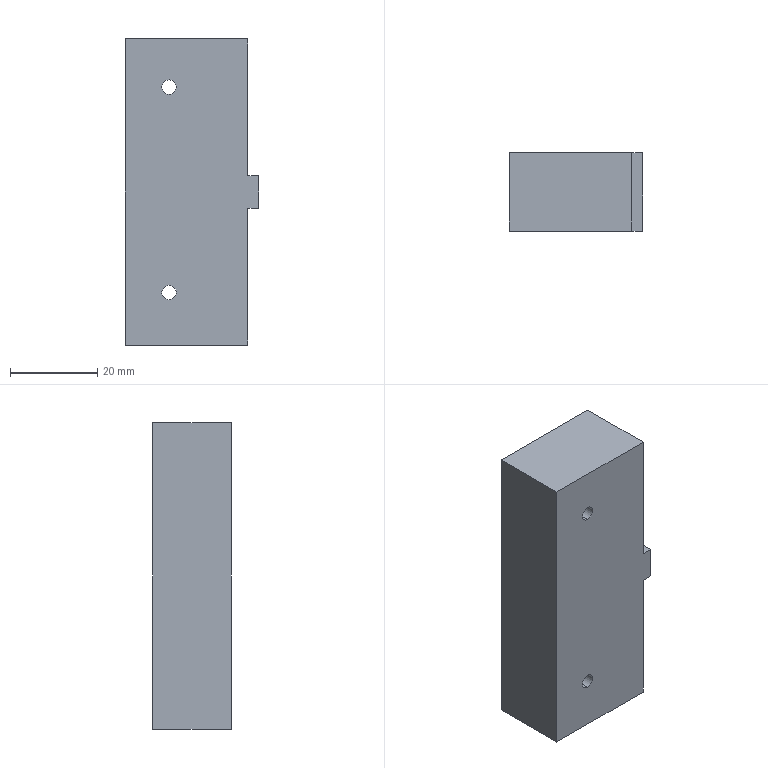Component | SolidWorks | CylinderFixingBlockS-1 | 1 solid | 22 faces | box 30.5 x 18 x 70 mm | volume 34906 mm3 | plane 10 | cylinder 8 | cone 4 | commonest cylinder face diameters 4.2 x4 3.3 x4
build123d program:
from build123d import *

# Parameters (mm, degrees)
SKETCH2_W             = 18
SKETCH2_H             = 28
BOSS_EXTRUDE1_DEPTH   = 70
M4_TAPPED_HOLE1_D     = 3.3
M5_TAPPED_HOLE1_D     = 4.2
M5_TAPPED_HOLE1_DEPTH = 14
M5_TAPPED_HOLE1_TIP   = 1.262
SKETCH8_W             = 7.4
SKETCH8_H             = 2.5
BOSS_EXTRUDE2_DEPTH   = 18


with BuildPart() as part:
    # Sketch2 → Boss-Extrude1 (new body)
    with BuildSketch(Plane.XY):
        with Locations((-28.849, -4)):
            Rectangle(SKETCH2_W, SKETCH2_H)
    extrude(amount=-BOSS_EXTRUDE1_DEPTH)

    # M4 Tapped Hole1 (through all)
    with Locations(Plane.ZY.offset(37.849)):
        with Locations((-11, 0), (-58, 0)):
            Hole(M4_TAPPED_HOLE1_D / 2)

    # M5 Tapped Hole1
    with Locations(Plane(origin=(0, -18, 0), x_dir=(-1, 0, 0), z_dir=(0, -1, 0))):
        with Locations((29.214, 58.5), (29.214, 11.5)):
            Hole(M5_TAPPED_HOLE1_D / 2, depth=M5_TAPPED_HOLE1_DEPTH)
            with Locations((0, 0, -(M5_TAPPED_HOLE1_DEPTH + M5_TAPPED_HOLE1_TIP / 2))):  # 118° drill point
                Cone(0, M5_TAPPED_HOLE1_D / 2, M5_TAPPED_HOLE1_TIP, mode=Mode.SUBTRACT)

    # Sketch8 → Boss-Extrude2 (add)
    with BuildSketch(Plane.ZY.offset(37.849)):
        with Locations((-35, -19.25)):
            Rectangle(SKETCH8_W, SKETCH8_H)
    extrude(amount=-BOSS_EXTRUDE2_DEPTH)


solid = part.part

# Placed as in the assembly
solid = solid.moved(Location((-524.996, 158.197, 306.626), (0, 0, 90)))
STEP:
#1=COLOUR_RGB('',0.7922,0.8196,0.9333);
#2=FILL_AREA_STYLE_COLOUR('',#1);
#3=FILL_AREA_STYLE('',(#2));
#4=SURFACE_STYLE_FILL_AREA(#3);
#5=SURFACE_SIDE_STYLE('',(#4));
#6=SURFACE_STYLE_USAGE(.BOTH.,#5);
#7=PRESENTATION_STYLE_ASSIGNMENT((#6));
#8=CARTESIAN_POINT('',(-20.512,5.078,9.851));
#9=VERTEX_POINT('',#8);
#10=CARTESIAN_POINT('',(-20.512,5.078,9.686));
#11=VERTEX_POINT('',#10);
#12=CARTESIAN_POINT('',(-20.512,5.078,9.769));
#13=DIRECTION('',(1.,-0.,-0.));
#14=DIRECTION('',(0.,0.,-1.));
#15=AXIS2_PLACEMENT_3D('',#12,#13,#14);
#16=CIRCLE('',#15,0.08268);
#17=EDGE_CURVE('',#9,#11,#16,.T.);
#18=ORIENTED_EDGE('',*,*,#17,.F.);
#19=CARTESIAN_POINT('',(-19.96,5.078,9.851));
#20=VERTEX_POINT('',#19);
#21=CARTESIAN_POINT('',(-19.96,5.078,9.851));
#22=DIRECTION('',(1.,-0.,-0.));
#23=VECTOR('',#22,39.37);
#24=LINE('',#21,#23);
#25=EDGE_CURVE('',#9,#20,#24,.T.);
#26=ORIENTED_EDGE('',*,*,#25,.T.);
#27=CARTESIAN_POINT('',(-19.96,5.078,9.686));
#28=VERTEX_POINT('',#27);
#29=CARTESIAN_POINT('',(-19.96,5.078,9.769));
#30=DIRECTION('',(1.,-0.,-0.));
#31=DIRECTION('',(0.,0.,-1.));
#32=AXIS2_PLACEMENT_3D('',#29,#30,#31);
#33=CIRCLE('',#32,0.08268);
#34=EDGE_CURVE('',#20,#28,#33,.T.);
#35=ORIENTED_EDGE('',*,*,#34,.T.);
#36=CARTESIAN_POINT('',(-19.96,5.078,9.686));
#37=DIRECTION('',(1.,-0.,-0.));
#38=VECTOR('',#37,39.37);
#39=LINE('',#36,#38);
#40=EDGE_CURVE('',#11,#28,#39,.T.);
#41=ORIENTED_EDGE('',*,*,#40,.F.);
#42=EDGE_LOOP('',(#18,#26,#35,#41));
#43=FACE_OUTER_BOUND('',#42,.T.);
#44=CARTESIAN_POINT('',(-19.96,5.078,9.769));
#45=DIRECTION('',(1.,-0.,-0.));
#46=DIRECTION('',(0.,0.,-1.));
#47=AXIS2_PLACEMENT_3D('',#44,#45,#46);
#48=CYLINDRICAL_SURFACE('',#47,0.08268);
#49=ADVANCED_FACE('',(#43),#48,.F.);
#50=CARTESIAN_POINT('',(-20.561,5.078,9.769));
#51=VERTEX_POINT('',#50);
#52=CARTESIAN_POINT('',(-20.512,5.078,9.686));
#53=DIRECTION('',(0.515,0.,-0.8572));
#54=VECTOR('',#53,39.37);
#55=LINE('',#52,#54);
#56=EDGE_CURVE('',#51,#11,#55,.T.);
#57=ORIENTED_EDGE('',*,*,#56,.F.);
#58=CARTESIAN_POINT('',(-20.512,5.078,9.851));
#59=DIRECTION('',(0.515,-0.,0.8572));
#60=VECTOR('',#59,39.37);
#61=LINE('',#58,#60);
#62=EDGE_CURVE('',#51,#9,#61,.T.);
#63=ORIENTED_EDGE('',*,*,#62,.T.);
#64=ORIENTED_EDGE('',*,*,#17,.T.);
#65=EDGE_LOOP('',(#57,#63,#64));
#66=FACE_OUTER_BOUND('',#65,.T.);
#67=CARTESIAN_POINT('',(-20.512,5.078,9.769));
#68=DIRECTION('',(1.,-0.,-0.));
#69=DIRECTION('',(0.,0.,-1.));
#70=AXIS2_PLACEMENT_3D('',#67,#68,#69);
#71=CONICAL_SURFACE('',#70,0.08268,1.03);
#72=ADVANCED_FACE('',(#66),#71,.F.);
#73=CARTESIAN_POINT('',(-20.512,5.078,11.702));
#74=VERTEX_POINT('',#73);
#75=CARTESIAN_POINT('',(-20.512,5.078,11.536));
#76=VERTEX_POINT('',#75);
#77=CARTESIAN_POINT('',(-20.512,5.078,11.619));
#78=DIRECTION('',(1.,-0.,-0.));
#79=DIRECTION('',(0.,0.,-1.));
#80=AXIS2_PLACEMENT_3D('',#77,#78,#79);
#81=CIRCLE('',#80,0.08268);
#82=EDGE_CURVE('',#74,#76,#81,.T.);
#83=ORIENTED_EDGE('',*,*,#82,.F.);
#84=CARTESIAN_POINT('',(-19.96,5.078,11.702));
#85=VERTEX_POINT('',#84);
#86=CARTESIAN_POINT('',(-19.96,5.078,11.702));
#87=DIRECTION('',(1.,-0.,-0.));
#88=VECTOR('',#87,39.37);
#89=LINE('',#86,#88);
#90=EDGE_CURVE('',#74,#85,#89,.T.);
#91=ORIENTED_EDGE('',*,*,#90,.T.);
#92=CARTESIAN_POINT('',(-19.96,5.078,11.536));
#93=VERTEX_POINT('',#92);
#94=CARTESIAN_POINT('',(-19.96,5.078,11.619));
#95=DIRECTION('',(1.,-0.,-0.));
#96=DIRECTION('',(0.,0.,-1.));
#97=AXIS2_PLACEMENT_3D('',#94,#95,#96);
#98=CIRCLE('',#97,0.08268);
#99=EDGE_CURVE('',#85,#93,#98,.T.);
#100=ORIENTED_EDGE('',*,*,#99,.T.);
#101=CARTESIAN_POINT('',(-19.96,5.078,11.536));
#102=DIRECTION('',(1.,-0.,-0.));
#103=VECTOR('',#102,39.37);
#104=LINE('',#101,#103);
#105=EDGE_CURVE('',#76,#93,#104,.T.);
#106=ORIENTED_EDGE('',*,*,#105,.F.);
#107=EDGE_LOOP('',(#83,#91,#100,#106));
#108=FACE_OUTER_BOUND('',#107,.T.);
#109=CARTESIAN_POINT('',(-19.96,5.078,11.619));
#110=DIRECTION('',(1.,-0.,-0.));
#111=DIRECTION('',(0.,0.,-1.));
#112=AXIS2_PLACEMENT_3D('',#109,#110,#111);
#113=CYLINDRICAL_SURFACE('',#112,0.08268);
#114=ADVANCED_FACE('',(#108),#113,.F.);
#115=CARTESIAN_POINT('',(-20.561,5.078,11.619));
#116=VERTEX_POINT('',#115);
#117=CARTESIAN_POINT('',(-20.512,5.078,11.536));
#118=DIRECTION('',(0.515,0.,-0.8572));
#119=VECTOR('',#118,39.37);
#120=LINE('',#117,#119);
#121=EDGE_CURVE('',#116,#76,#120,.T.);
#122=ORIENTED_EDGE('',*,*,#121,.F.);
#123=CARTESIAN_POINT('',(-20.512,5.078,11.702));
#124=DIRECTION('',(0.515,-0.,0.8572));
#125=VECTOR('',#124,39.37);
#126=LINE('',#123,#125);
#127=EDGE_CURVE('',#116,#74,#126,.T.);
#128=ORIENTED_EDGE('',*,*,#127,.T.);
#129=ORIENTED_EDGE('',*,*,#82,.T.);
#130=EDGE_LOOP('',(#122,#128,#129));
#131=FACE_OUTER_BOUND('',#130,.T.);
#132=CARTESIAN_POINT('',(-20.512,5.078,11.619));
#133=DIRECTION('',(1.,-0.,-0.));
#134=DIRECTION('',(0.,0.,-1.));
#135=AXIS2_PLACEMENT_3D('',#132,#133,#134);
#136=CONICAL_SURFACE('',#135,0.08268,1.03);
#137=ADVANCED_FACE('',(#131),#136,.F.);
#138=CARTESIAN_POINT('',(-20.669,5.447,11.574));
#139=VERTEX_POINT('',#138);
#140=CARTESIAN_POINT('',(-20.669,5.447,11.704));
#141=VERTEX_POINT('',#140);
#142=CARTESIAN_POINT('',(-20.669,5.447,11.639));
#143=DIRECTION('',(0.,-1.,-0.));
#144=DIRECTION('',(0.,0.,1.));
#145=AXIS2_PLACEMENT_3D('',#142,#143,#144);
#146=CIRCLE('',#145,0.06496);
#147=EDGE_CURVE('',#139,#141,#146,.T.);
#148=ORIENTED_EDGE('',*,*,#147,.F.);
#149=CARTESIAN_POINT('',(-20.669,4.738,11.574));
#150=VERTEX_POINT('',#149);
#151=CARTESIAN_POINT('',(-20.669,4.738,11.574));
#152=DIRECTION('',(0.,-1.,-0.));
#153=VECTOR('',#152,39.37);
#154=LINE('',#151,#153);
#155=EDGE_CURVE('',#139,#150,#154,.T.);
#156=ORIENTED_EDGE('',*,*,#155,.T.);
#157=CARTESIAN_POINT('',(-20.669,4.738,11.704));
#158=VERTEX_POINT('',#157);
#159=CARTESIAN_POINT('',(-20.669,4.738,11.639));
#160=DIRECTION('',(0.,-1.,-0.));
#161=DIRECTION('',(0.,0.,1.));
#162=AXIS2_PLACEMENT_3D('',#159,#160,#161);
#163=CIRCLE('',#162,0.06496);
#164=EDGE_CURVE('',#150,#158,#163,.T.);
#165=ORIENTED_EDGE('',*,*,#164,.T.);
#166=CARTESIAN_POINT('',(-20.669,4.738,11.704));
#167=DIRECTION('',(0.,-1.,-0.));
#168=VECTOR('',#167,39.37);
#169=LINE('',#166,#168);
#170=EDGE_CURVE('',#141,#158,#169,.T.);
#171=ORIENTED_EDGE('',*,*,#170,.F.);
#172=EDGE_LOOP('',(#148,#156,#165,#171));
#173=FACE_OUTER_BOUND('',#172,.T.);
#174=CARTESIAN_POINT('',(-20.669,4.738,11.639));
#175=DIRECTION('',(0.,-1.,-0.));
#176=DIRECTION('',(0.,0.,1.));
#177=AXIS2_PLACEMENT_3D('',#174,#175,#176);
#178=CYLINDRICAL_SURFACE('',#177,0.06496);
#179=ADVANCED_FACE('',(#173),#178,.F.);
#180=CARTESIAN_POINT('',(-20.669,5.447,9.723));
#181=VERTEX_POINT('',#180);
#182=CARTESIAN_POINT('',(-20.669,5.447,9.853));
#183=VERTEX_POINT('',#182);
#184=CARTESIAN_POINT('',(-20.669,5.447,9.788));
#185=DIRECTION('',(0.,-1.,-0.));
#186=DIRECTION('',(0.,0.,1.));
#187=AXIS2_PLACEMENT_3D('',#184,#185,#186);
#188=CIRCLE('',#187,0.06496);
#189=EDGE_CURVE('',#181,#183,#188,.T.);
#190=ORIENTED_EDGE('',*,*,#189,.F.);
#191=CARTESIAN_POINT('',(-20.669,4.738,9.723));
#192=VERTEX_POINT('',#191);
#193=CARTESIAN_POINT('',(-20.669,4.738,9.723));
#194=DIRECTION('',(0.,-1.,-0.));
#195=VECTOR('',#194,39.37);
#196=LINE('',#193,#195);
#197=EDGE_CURVE('',#181,#192,#196,.T.);
#198=ORIENTED_EDGE('',*,*,#197,.T.);
#199=CARTESIAN_POINT('',(-20.669,4.738,9.853));
#200=VERTEX_POINT('',#199);
#201=CARTESIAN_POINT('',(-20.669,4.738,9.788));
#202=DIRECTION('',(0.,-1.,-0.));
#203=DIRECTION('',(0.,0.,1.));
#204=AXIS2_PLACEMENT_3D('',#201,#202,#203);
#205=CIRCLE('',#204,0.06496);
#206=EDGE_CURVE('',#192,#200,#205,.T.);
#207=ORIENTED_EDGE('',*,*,#206,.T.);
#208=CARTESIAN_POINT('',(-20.669,4.738,9.853));
#209=DIRECTION('',(0.,-1.,-0.));
#210=VECTOR('',#209,39.37);
#211=LINE('',#208,#210);
#212=EDGE_CURVE('',#183,#200,#211,.T.);
#213=ORIENTED_EDGE('',*,*,#212,.F.);
#214=EDGE_LOOP('',(#190,#198,#207,#213));
#215=FACE_OUTER_BOUND('',#214,.T.);
#216=CARTESIAN_POINT('',(-20.669,4.738,9.788));
#217=DIRECTION('',(0.,-1.,-0.));
#218=DIRECTION('',(0.,0.,1.));
#219=AXIS2_PLACEMENT_3D('',#216,#217,#218);
#220=CYLINDRICAL_SURFACE('',#219,0.06496);
#221=ADVANCED_FACE('',(#215),#220,.F.);
#222=CARTESIAN_POINT('',(-19.96,5.078,9.769));
#223=DIRECTION('',(1.,-0.,-0.));
#224=DIRECTION('',(0.,0.,-1.));
#225=AXIS2_PLACEMENT_3D('',#222,#223,#224);
#226=CIRCLE('',#225,0.08268);
#227=EDGE_CURVE('',#28,#20,#226,.T.);
#228=ORIENTED_EDGE('',*,*,#227,.F.);
#229=ORIENTED_EDGE('',*,*,#34,.F.);
#230=EDGE_LOOP('',(#228,#229));
#231=FACE_BOUND('',#230,.T.);
#232=CARTESIAN_POINT('',(-19.96,5.447,9.316));
#233=VERTEX_POINT('',#232);
#234=CARTESIAN_POINT('',(-19.96,5.447,10.548));
#235=VERTEX_POINT('',#234);
#236=CARTESIAN_POINT('',(-19.96,5.447,9.316));
#237=DIRECTION('',(0.,-0.,1.));
#238=VECTOR('',#237,39.37);
#239=LINE('',#236,#238);
#240=EDGE_CURVE('',#233,#235,#239,.T.);
#241=ORIENTED_EDGE('',*,*,#240,.T.);
#242=CARTESIAN_POINT('',(-19.96,4.738,10.548));
#243=VERTEX_POINT('',#242);
#244=CARTESIAN_POINT('',(-19.96,5.754,10.548));
#245=DIRECTION('',(0.,-1.,-0.));
#246=VECTOR('',#245,39.37);
#247=LINE('',#244,#246);
#248=EDGE_CURVE('',#235,#243,#247,.T.);
#249=ORIENTED_EDGE('',*,*,#248,.T.);
#250=CARTESIAN_POINT('',(-19.96,4.738,9.316));
#251=VERTEX_POINT('',#250);
#252=CARTESIAN_POINT('',(-19.96,4.738,9.316));
#253=DIRECTION('',(0.,-0.,1.));
#254=VECTOR('',#253,39.37);
#255=LINE('',#252,#254);
#256=EDGE_CURVE('',#251,#243,#255,.T.);
#257=ORIENTED_EDGE('',*,*,#256,.F.);
#258=CARTESIAN_POINT('',(-19.96,4.738,9.316));
#259=DIRECTION('',(-0.,1.,0.));
#260=VECTOR('',#259,39.37);
#261=LINE('',#258,#260);
#262=EDGE_CURVE('',#251,#233,#261,.T.);
#263=ORIENTED_EDGE('',*,*,#262,.T.);
#264=EDGE_LOOP('',(#241,#249,#257,#263));
#265=FACE_OUTER_BOUND('',#264,.T.);
#266=CARTESIAN_POINT('',(-19.96,4.738,9.316));
#267=DIRECTION('',(1.,-0.,-0.));
#268=DIRECTION('',(-0.,0.,-1.));
#269=AXIS2_PLACEMENT_3D('',#266,#267,#268);
#270=PLANE('',#269);
#271=ADVANCED_FACE('',(#231,#265),#270,.T.);
#272=CARTESIAN_POINT('',(-20.669,4.738,11.639));
#273=DIRECTION('',(0.,-1.,-0.));
#274=DIRECTION('',(0.,0.,1.));
#275=AXIS2_PLACEMENT_3D('',#272,#273,#274);
#276=CIRCLE('',#275,0.06496);
#277=EDGE_CURVE('',#158,#150,#276,.T.);
#278=ORIENTED_EDGE('',*,*,#277,.F.);
#279=ORIENTED_EDGE('',*,*,#164,.F.);
#280=EDGE_LOOP('',(#278,#279));
#281=FACE_BOUND('',#280,.T.);
#282=CARTESIAN_POINT('',(-20.669,4.738,9.788));
#283=DIRECTION('',(0.,-1.,-0.));
#284=DIRECTION('',(0.,0.,1.));
#285=AXIS2_PLACEMENT_3D('',#282,#283,#284);
#286=CIRCLE('',#285,0.06496);
#287=EDGE_CURVE('',#200,#192,#286,.T.);
#288=ORIENTED_EDGE('',*,*,#287,.F.);
#289=ORIENTED_EDGE('',*,*,#206,.F.);
#290=EDGE_LOOP('',(#288,#289));
#291=FACE_BOUND('',#290,.T.);
#292=CARTESIAN_POINT('',(-21.063,4.738,12.072));
#293=VERTEX_POINT('',#292);
#294=CARTESIAN_POINT('',(-19.96,4.738,12.072));
#295=VERTEX_POINT('',#294);
#296=CARTESIAN_POINT('',(-21.063,4.738,12.072));
#297=DIRECTION('',(1.,-0.,-0.));
#298=VECTOR('',#297,39.37);
#299=LINE('',#296,#298);
#300=EDGE_CURVE('',#293,#295,#299,.T.);
#301=ORIENTED_EDGE('',*,*,#300,.F.);
#302=CARTESIAN_POINT('',(-21.063,4.738,9.316));
#303=VERTEX_POINT('',#302);
#304=CARTESIAN_POINT('',(-21.063,4.738,9.316));
#305=DIRECTION('',(0.,-0.,1.));
#306=VECTOR('',#305,39.37);
#307=LINE('',#304,#306);
#308=EDGE_CURVE('',#303,#293,#307,.T.);
#309=ORIENTED_EDGE('',*,*,#308,.F.);
#310=CARTESIAN_POINT('',(-21.063,4.738,9.316));
#311=DIRECTION('',(1.,-0.,-0.));
#312=VECTOR('',#311,39.37);
#313=LINE('',#310,#312);
#314=EDGE_CURVE('',#303,#251,#313,.T.);
#315=ORIENTED_EDGE('',*,*,#314,.T.);
#316=ORIENTED_EDGE('',*,*,#256,.T.);
#317=CARTESIAN_POINT('',(-19.862,4.738,10.548));
#318=VERTEX_POINT('',#317);
#319=CARTESIAN_POINT('',(-19.96,4.738,10.548));
#320=DIRECTION('',(1.,-0.,-0.));
#321=VECTOR('',#320,39.37);
#322=LINE('',#319,#321);
#323=EDGE_CURVE('',#243,#318,#322,.T.);
#324=ORIENTED_EDGE('',*,*,#323,.T.);
#325=CARTESIAN_POINT('',(-19.862,4.738,10.84));
#326=VERTEX_POINT('',#325);
#327=CARTESIAN_POINT('',(-19.862,4.738,10.84));
#328=DIRECTION('',(0.,-0.,1.));
#329=VECTOR('',#328,39.37);
#330=LINE('',#327,#329);
#331=EDGE_CURVE('',#318,#326,#330,.T.);
#332=ORIENTED_EDGE('',*,*,#331,.T.);
#333=CARTESIAN_POINT('',(-19.96,4.738,10.84));
#334=VERTEX_POINT('',#333);
#335=CARTESIAN_POINT('',(-19.96,4.738,10.84));
#336=DIRECTION('',(-1.,0.,0.));
#337=VECTOR('',#336,39.37);
#338=LINE('',#335,#337);
#339=EDGE_CURVE('',#326,#334,#338,.T.);
#340=ORIENTED_EDGE('',*,*,#339,.T.);
#341=CARTESIAN_POINT('',(-19.96,4.738,9.316));
#342=DIRECTION('',(0.,-0.,1.));
#343=VECTOR('',#342,39.37);
#344=LINE('',#341,#343);
#345=EDGE_CURVE('',#334,#295,#344,.T.);
#346=ORIENTED_EDGE('',*,*,#345,.T.);
#347=EDGE_LOOP('',(#301,#309,#315,#316,#324,#332,#340,#346));
#348=FACE_OUTER_BOUND('',#347,.T.);
#349=CARTESIAN_POINT('',(-21.063,4.738,9.316));
#350=DIRECTION('',(0.,-1.,-0.));
#351=DIRECTION('',(0.,-0.,1.));
#352=AXIS2_PLACEMENT_3D('',#349,#350,#351);
#353=PLANE('',#352);
#354=ADVANCED_FACE('',(#281,#291,#348),#353,.T.);
#355=CARTESIAN_POINT('',(-21.063,5.447,12.072));
#356=VERTEX_POINT('',#355);
#357=CARTESIAN_POINT('',(-21.063,4.738,12.072));
#358=DIRECTION('',(0.,-1.,-0.));
#359=VECTOR('',#358,39.37);
#360=LINE('',#357,#359);
#361=EDGE_CURVE('',#356,#293,#360,.T.);
#362=ORIENTED_EDGE('',*,*,#361,.F.);
#363=CARTESIAN_POINT('',(-21.063,5.447,9.316));
#364=VERTEX_POINT('',#363);
#365=CARTESIAN_POINT('',(-21.063,5.447,9.316));
#366=DIRECTION('',(0.,-0.,1.));
#367=VECTOR('',#366,39.37);
#368=LINE('',#365,#367);
#369=EDGE_CURVE('',#364,#356,#368,.T.);
#370=ORIENTED_EDGE('',*,*,#369,.F.);
#371=CARTESIAN_POINT('',(-21.063,4.738,9.316));
#372=DIRECTION('',(0.,-1.,-0.));
#373=VECTOR('',#372,39.37);
#374=LINE('',#371,#373);
#375=EDGE_CURVE('',#364,#303,#374,.T.);
#376=ORIENTED_EDGE('',*,*,#375,.T.);
#377=ORIENTED_EDGE('',*,*,#308,.T.);
#378=EDGE_LOOP('',(#362,#370,#376,#377));
#379=FACE_OUTER_BOUND('',#378,.T.);
#380=CARTESIAN_POINT('',(-21.063,4.738,9.316));
#381=DIRECTION('',(-1.,0.,0.));
#382=DIRECTION('',(0.,-0.,1.));
#383=AXIS2_PLACEMENT_3D('',#380,#381,#382);
#384=PLANE('',#383);
#385=ADVANCED_FACE('',(#379),#384,.T.);
#386=CARTESIAN_POINT('',(-20.669,5.447,11.639));
#387=DIRECTION('',(0.,-1.,-0.));
#388=DIRECTION('',(0.,0.,1.));
#389=AXIS2_PLACEMENT_3D('',#386,#387,#388);
#390=CIRCLE('',#389,0.06496);
#391=EDGE_CURVE('',#141,#139,#390,.T.);
#392=ORIENTED_EDGE('',*,*,#391,.T.);
#393=ORIENTED_EDGE('',*,*,#147,.T.);
#394=EDGE_LOOP('',(#392,#393));
#395=FACE_BOUND('',#394,.T.);
#396=CARTESIAN_POINT('',(-20.669,5.447,9.788));
#397=DIRECTION('',(0.,-1.,-0.));
#398=DIRECTION('',(0.,0.,1.));
#399=AXIS2_PLACEMENT_3D('',#396,#397,#398);
#400=CIRCLE('',#399,0.06496);
#401=EDGE_CURVE('',#183,#181,#400,.T.);
#402=ORIENTED_EDGE('',*,*,#401,.T.);
#403=ORIENTED_EDGE('',*,*,#189,.T.);
#404=EDGE_LOOP('',(#402,#403));
#405=FACE_BOUND('',#404,.T.);
#406=CARTESIAN_POINT('',(-19.96,5.447,12.072));
#407=VERTEX_POINT('',#406);
#408=CARTESIAN_POINT('',(-21.063,5.447,12.072));
#409=DIRECTION('',(-1.,-0.,0.));
#410=VECTOR('',#409,39.37);
#411=LINE('',#408,#410);
#412=EDGE_CURVE('',#407,#356,#411,.T.);
#413=ORIENTED_EDGE('',*,*,#412,.F.);
#414=CARTESIAN_POINT('',(-19.96,5.447,10.84));
#415=VERTEX_POINT('',#414);
#416=CARTESIAN_POINT('',(-19.96,5.447,9.316));
#417=DIRECTION('',(0.,-0.,1.));
#418=VECTOR('',#417,39.37);
#419=LINE('',#416,#418);
#420=EDGE_CURVE('',#415,#407,#419,.T.);
#421=ORIENTED_EDGE('',*,*,#420,.F.);
#422=CARTESIAN_POINT('',(-19.862,5.447,10.84));
#423=VERTEX_POINT('',#422);
#424=CARTESIAN_POINT('',(-19.96,5.447,10.84));
#425=DIRECTION('',(-1.,-0.,0.));
#426=VECTOR('',#425,39.37);
#427=LINE('',#424,#426);
#428=EDGE_CURVE('',#423,#415,#427,.T.);
#429=ORIENTED_EDGE('',*,*,#428,.F.);
#430=CARTESIAN_POINT('',(-19.862,5.447,10.548));
#431=VERTEX_POINT('',#430);
#432=CARTESIAN_POINT('',(-19.862,5.447,10.84));
#433=DIRECTION('',(0.,-0.,1.));
#434=VECTOR('',#433,39.37);
#435=LINE('',#432,#434);
#436=EDGE_CURVE('',#431,#423,#435,.T.);
#437=ORIENTED_EDGE('',*,*,#436,.F.);
#438=CARTESIAN_POINT('',(-19.96,5.447,10.548));
#439=DIRECTION('',(1.,0.,-0.));
#440=VECTOR('',#439,39.37);
#441=LINE('',#438,#440);
#442=EDGE_CURVE('',#235,#431,#441,.T.);
#443=ORIENTED_EDGE('',*,*,#442,.F.);
#444=ORIENTED_EDGE('',*,*,#240,.F.);
#445=CARTESIAN_POINT('',(-21.063,5.447,9.316));
#446=DIRECTION('',(-1.,-0.,0.));
#447=VECTOR('',#446,39.37);
#448=LINE('',#445,#447);
#449=EDGE_CURVE('',#233,#364,#448,.T.);
#450=ORIENTED_EDGE('',*,*,#449,.T.);
#451=ORIENTED_EDGE('',*,*,#369,.T.);
#452=EDGE_LOOP('',(#413,#421,#429,#437,#443,#444,#450,#451));
#453=FACE_OUTER_BOUND('',#452,.T.);
#454=CARTESIAN_POINT('',(-21.063,5.447,9.316));
#455=DIRECTION('',(-0.,1.,0.));
#456=DIRECTION('',(-1.,-0.,0.));
#457=AXIS2_PLACEMENT_3D('',#454,#455,#456);
#458=PLANE('',#457);
#459=ADVANCED_FACE('',(#395,#405,#453),#458,.T.);
#460=CARTESIAN_POINT('',(-19.96,5.754,10.84));
#461=DIRECTION('',(0.,-1.,-0.));
#462=VECTOR('',#461,39.37);
#463=LINE('',#460,#462);
#464=EDGE_CURVE('',#415,#334,#463,.T.);
#465=ORIENTED_EDGE('',*,*,#464,.F.);
#466=ORIENTED_EDGE('',*,*,#420,.T.);
#467=CARTESIAN_POINT('',(-19.96,4.738,12.072));
#468=DIRECTION('',(-0.,1.,0.));
#469=VECTOR('',#468,39.37);
#470=LINE('',#467,#469);
#471=EDGE_CURVE('',#295,#407,#470,.T.);
#472=ORIENTED_EDGE('',*,*,#471,.F.);
#473=ORIENTED_EDGE('',*,*,#345,.F.);
#474=EDGE_LOOP('',(#465,#466,#472,#473));
#475=FACE_OUTER_BOUND('',#474,.T.);
#476=CARTESIAN_POINT('',(-19.96,5.078,11.619));
#477=DIRECTION('',(1.,-0.,-0.));
#478=DIRECTION('',(0.,0.,-1.));
#479=AXIS2_PLACEMENT_3D('',#476,#477,#478);
#480=CIRCLE('',#479,0.08268);
#481=EDGE_CURVE('',#93,#85,#480,.T.);
#482=ORIENTED_EDGE('',*,*,#481,.F.);
#483=ORIENTED_EDGE('',*,*,#99,.F.);
#484=EDGE_LOOP('',(#482,#483));
#485=FACE_BOUND('',#484,.T.);
#486=CARTESIAN_POINT('',(-19.96,4.738,9.316));
#487=DIRECTION('',(1.,-0.,-0.));
#488=DIRECTION('',(-0.,0.,-1.));
#489=AXIS2_PLACEMENT_3D('',#486,#487,#488);
#490=PLANE('',#489);
#491=ADVANCED_FACE('',(#475,#485),#490,.T.);
#492=ORIENTED_EDGE('',*,*,#314,.F.);
#493=ORIENTED_EDGE('',*,*,#375,.F.);
#494=ORIENTED_EDGE('',*,*,#449,.F.);
#495=ORIENTED_EDGE('',*,*,#262,.F.);
#496=EDGE_LOOP('',(#492,#493,#494,#495));
#497=FACE_OUTER_BOUND('',#496,.T.);
#498=CARTESIAN_POINT('',(-20.669,6.228,9.316));
#499=DIRECTION('',(0.,-0.,1.));
#500=DIRECTION('',(-0.,1.,0.));
#501=AXIS2_PLACEMENT_3D('',#498,#499,#500);
#502=PLANE('',#501);
#503=ADVANCED_FACE('',(#497),#502,.F.);
#504=ORIENTED_EDGE('',*,*,#300,.T.);
#505=ORIENTED_EDGE('',*,*,#471,.T.);
#506=ORIENTED_EDGE('',*,*,#412,.T.);
#507=ORIENTED_EDGE('',*,*,#361,.T.);
#508=EDGE_LOOP('',(#504,#505,#506,#507));
#509=FACE_OUTER_BOUND('',#508,.T.);
#510=CARTESIAN_POINT('',(-20.669,6.228,12.072));
#511=DIRECTION('',(0.,-0.,1.));
#512=DIRECTION('',(-0.,1.,0.));
#513=AXIS2_PLACEMENT_3D('',#510,#511,#512);
#514=PLANE('',#513);
#515=ADVANCED_FACE('',(#509),#514,.T.);
#516=ORIENTED_EDGE('',*,*,#197,.F.);
#517=ORIENTED_EDGE('',*,*,#401,.F.);
#518=ORIENTED_EDGE('',*,*,#212,.T.);
#519=ORIENTED_EDGE('',*,*,#287,.T.);
#520=EDGE_LOOP('',(#516,#517,#518,#519));
#521=FACE_OUTER_BOUND('',#520,.T.);
#522=CARTESIAN_POINT('',(-20.669,4.738,9.788));
#523=DIRECTION('',(0.,-1.,-0.));
#524=DIRECTION('',(0.,0.,1.));
#525=AXIS2_PLACEMENT_3D('',#522,#523,#524);
#526=CYLINDRICAL_SURFACE('',#525,0.06496);
#527=ADVANCED_FACE('',(#521),#526,.F.);
#528=ORIENTED_EDGE('',*,*,#155,.F.);
#529=ORIENTED_EDGE('',*,*,#391,.F.);
#530=ORIENTED_EDGE('',*,*,#170,.T.);
#531=ORIENTED_EDGE('',*,*,#277,.T.);
#532=EDGE_LOOP('',(#528,#529,#530,#531));
#533=FACE_OUTER_BOUND('',#532,.T.);
#534=CARTESIAN_POINT('',(-20.669,4.738,11.639));
#535=DIRECTION('',(0.,-1.,-0.));
#536=DIRECTION('',(0.,0.,1.));
#537=AXIS2_PLACEMENT_3D('',#534,#535,#536);
#538=CYLINDRICAL_SURFACE('',#537,0.06496);
#539=ADVANCED_FACE('',(#533),#538,.F.);
#540=ORIENTED_EDGE('',*,*,#127,.F.);
#541=ORIENTED_EDGE('',*,*,#121,.T.);
#542=CARTESIAN_POINT('',(-20.512,5.078,11.619));
#543=DIRECTION('',(1.,-0.,-0.));
#544=DIRECTION('',(0.,0.,-1.));
#545=AXIS2_PLACEMENT_3D('',#542,#543,#544);
#546=CIRCLE('',#545,0.08268);
#547=EDGE_CURVE('',#76,#74,#546,.T.);
#548=ORIENTED_EDGE('',*,*,#547,.T.);
#549=EDGE_LOOP('',(#540,#541,#548));
#550=FACE_OUTER_BOUND('',#549,.T.);
#551=CARTESIAN_POINT('',(-20.512,5.078,11.619));
#552=DIRECTION('',(1.,-0.,-0.));
#553=DIRECTION('',(0.,0.,-1.));
#554=AXIS2_PLACEMENT_3D('',#551,#552,#553);
#555=CONICAL_SURFACE('',#554,0.08268,1.03);
#556=ADVANCED_FACE('',(#550),#555,.F.);
#557=ORIENTED_EDGE('',*,*,#90,.F.);
#558=ORIENTED_EDGE('',*,*,#547,.F.);
#559=ORIENTED_EDGE('',*,*,#105,.T.);
#560=ORIENTED_EDGE('',*,*,#481,.T.);
#561=EDGE_LOOP('',(#557,#558,#559,#560));
#562=FACE_OUTER_BOUND('',#561,.T.);
#563=CARTESIAN_POINT('',(-19.96,5.078,11.619));
#564=DIRECTION('',(1.,-0.,-0.));
#565=DIRECTION('',(0.,0.,-1.));
#566=AXIS2_PLACEMENT_3D('',#563,#564,#565);
#567=CYLINDRICAL_SURFACE('',#566,0.08268);
#568=ADVANCED_FACE('',(#562),#567,.F.);
#569=ORIENTED_EDGE('',*,*,#62,.F.);
#570=ORIENTED_EDGE('',*,*,#56,.T.);
#571=CARTESIAN_POINT('',(-20.512,5.078,9.769));
#572=DIRECTION('',(1.,-0.,-0.));
#573=DIRECTION('',(0.,0.,-1.));
#574=AXIS2_PLACEMENT_3D('',#571,#572,#573);
#575=CIRCLE('',#574,0.08268);
#576=EDGE_CURVE('',#11,#9,#575,.T.);
#577=ORIENTED_EDGE('',*,*,#576,.T.);
#578=EDGE_LOOP('',(#569,#570,#577));
#579=FACE_OUTER_BOUND('',#578,.T.);
#580=CARTESIAN_POINT('',(-20.512,5.078,9.769));
#581=DIRECTION('',(1.,-0.,-0.));
#582=DIRECTION('',(0.,0.,-1.));
#583=AXIS2_PLACEMENT_3D('',#580,#581,#582);
#584=CONICAL_SURFACE('',#583,0.08268,1.03);
#585=ADVANCED_FACE('',(#579),#584,.F.);
#586=ORIENTED_EDGE('',*,*,#25,.F.);
#587=ORIENTED_EDGE('',*,*,#576,.F.);
#588=ORIENTED_EDGE('',*,*,#40,.T.);
#589=ORIENTED_EDGE('',*,*,#227,.T.);
#590=EDGE_LOOP('',(#586,#587,#588,#589));
#591=FACE_OUTER_BOUND('',#590,.T.);
#592=CARTESIAN_POINT('',(-19.96,5.078,9.769));
#593=DIRECTION('',(1.,-0.,-0.));
#594=DIRECTION('',(0.,0.,-1.));
#595=AXIS2_PLACEMENT_3D('',#592,#593,#594);
#596=CYLINDRICAL_SURFACE('',#595,0.08268);
#597=ADVANCED_FACE('',(#591),#596,.F.);
#598=ORIENTED_EDGE('',*,*,#248,.F.);
#599=ORIENTED_EDGE('',*,*,#442,.T.);
#600=CARTESIAN_POINT('',(-19.862,5.754,10.548));
#601=DIRECTION('',(0.,-1.,-0.));
#602=VECTOR('',#601,39.37);
#603=LINE('',#600,#602);
#604=EDGE_CURVE('',#431,#318,#603,.T.);
#605=ORIENTED_EDGE('',*,*,#604,.T.);
#606=ORIENTED_EDGE('',*,*,#323,.F.);
#607=EDGE_LOOP('',(#598,#599,#605,#606));
#608=FACE_OUTER_BOUND('',#607,.T.);
#609=CARTESIAN_POINT('',(-19.96,5.754,10.548));
#610=DIRECTION('',(-0.,0.,-1.));
#611=DIRECTION('',(0.,-1.,-0.));
#612=AXIS2_PLACEMENT_3D('',#609,#610,#611);
#613=PLANE('',#612);
#614=ADVANCED_FACE('',(#608),#613,.T.);
#615=ORIENTED_EDGE('',*,*,#604,.F.);
#616=ORIENTED_EDGE('',*,*,#436,.T.);
#617=CARTESIAN_POINT('',(-19.862,5.754,10.84));
#618=DIRECTION('',(0.,-1.,-0.));
#619=VECTOR('',#618,39.37);
#620=LINE('',#617,#619);
#621=EDGE_CURVE('',#423,#326,#620,.T.);
#622=ORIENTED_EDGE('',*,*,#621,.T.);
#623=ORIENTED_EDGE('',*,*,#331,.F.);
#624=EDGE_LOOP('',(#615,#616,#622,#623));
#625=FACE_OUTER_BOUND('',#624,.T.);
#626=CARTESIAN_POINT('',(-19.862,5.754,10.84));
#627=DIRECTION('',(1.,-0.,-0.));
#628=DIRECTION('',(-0.,0.,-1.));
#629=AXIS2_PLACEMENT_3D('',#626,#627,#628);
#630=PLANE('',#629);
#631=ADVANCED_FACE('',(#625),#630,.T.);
#632=ORIENTED_EDGE('',*,*,#621,.F.);
#633=ORIENTED_EDGE('',*,*,#428,.T.);
#634=ORIENTED_EDGE('',*,*,#464,.T.);
#635=ORIENTED_EDGE('',*,*,#339,.F.);
#636=EDGE_LOOP('',(#632,#633,#634,#635));
#637=FACE_OUTER_BOUND('',#636,.T.);
#638=CARTESIAN_POINT('',(-19.96,5.754,10.84));
#639=DIRECTION('',(0.,-0.,1.));
#640=DIRECTION('',(-0.,1.,0.));
#641=AXIS2_PLACEMENT_3D('',#638,#639,#640);
#642=PLANE('',#641);
#643=ADVANCED_FACE('',(#637),#642,.T.);
#644=CLOSED_SHELL('',(#49,#72,#114,#137,#179,#221,#271,#354,#385,#459,#491,#503,#515,#527,#539,#556,#568,#585,#597,#614,#631,#643));
#645=MANIFOLD_SOLID_BREP('',#644);
#646=STYLED_ITEM('',(#7),#645);
#647=PRESENTATION_LAYER_ASSIGNMENT('','',(#646));
#648=CARTESIAN_POINT('',(0.,0.,0.));
#649=DIRECTION('',(0.,0.,1.));
#650=DIRECTION('',(1.,0.,0.));
#651=AXIS2_PLACEMENT_3D('',#648,#649,#650);
#652=(LENGTH_UNIT()NAMED_UNIT(*)SI_UNIT($,.METRE.));
#653=LENGTH_MEASURE_WITH_UNIT(LENGTH_MEASURE(0.0254),#652);
#654=DIMENSIONAL_EXPONENTS(1.,0.,0.,0.,0.,0.,0.);
#655=(CONVERSION_BASED_UNIT('',#653)LENGTH_UNIT()NAMED_UNIT(#654));
#656=UNCERTAINTY_MEASURE_WITH_UNIT(LENGTH_MEASURE(0.00001),#655,'','');
#657=(NAMED_UNIT(*)PLANE_ANGLE_UNIT()SI_UNIT($,.RADIAN.));
#658=(NAMED_UNIT(*)SI_UNIT($,.STERADIAN.)SOLID_ANGLE_UNIT());
#659=(GEOMETRIC_REPRESENTATION_CONTEXT(3)GLOBAL_UNCERTAINTY_ASSIGNED_CONTEXT((#656))GLOBAL_UNIT_ASSIGNED_CONTEXT((#655,#657,#658))REPRESENTATION_CONTEXT('',''));
#660=ADVANCED_BREP_SHAPE_REPRESENTATION('',(#645,#651),#659);
#661=(LENGTH_UNIT()NAMED_UNIT(*)SI_UNIT($,.METRE.));
#662=LENGTH_MEASURE_WITH_UNIT(LENGTH_MEASURE(0.0254),#661);
#663=DIMENSIONAL_EXPONENTS(1.,0.,0.,0.,0.,0.,0.);
#664=(CONVERSION_BASED_UNIT('',#662)LENGTH_UNIT()NAMED_UNIT(#663));
#665=UNCERTAINTY_MEASURE_WITH_UNIT(LENGTH_MEASURE(0.00001),#664,'','');
#666=(NAMED_UNIT(*)PLANE_ANGLE_UNIT()SI_UNIT($,.RADIAN.));
#667=(NAMED_UNIT(*)SI_UNIT($,.STERADIAN.)SOLID_ANGLE_UNIT());
#668=(GEOMETRIC_REPRESENTATION_CONTEXT(3)GLOBAL_UNCERTAINTY_ASSIGNED_CONTEXT((#665))GLOBAL_UNIT_ASSIGNED_CONTEXT((#664,#666,#667))REPRESENTATION_CONTEXT('',''));
#669=MECHANICAL_DESIGN_GEOMETRIC_PRESENTATION_REPRESENTATION('',(#646),#668);